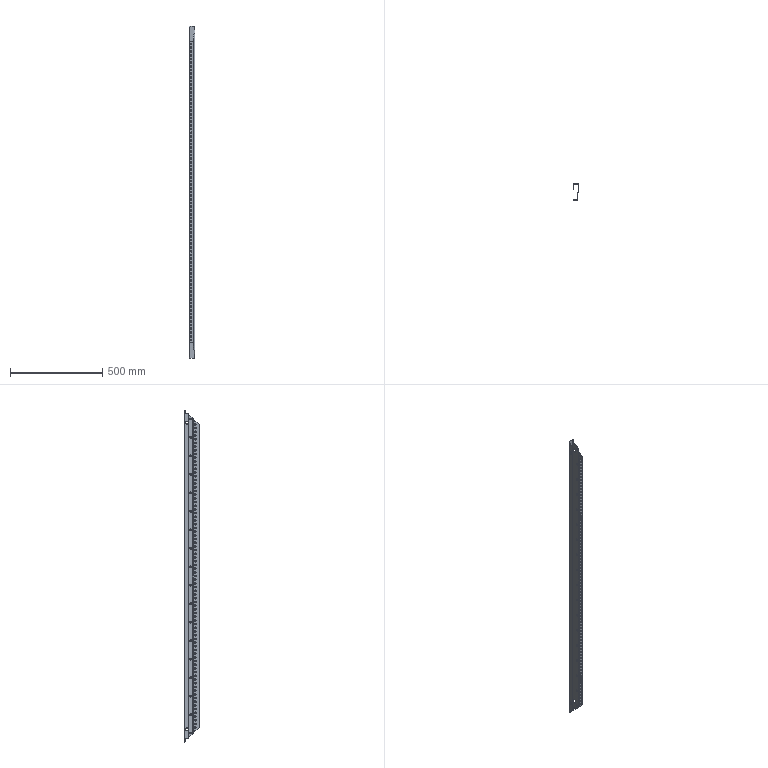Component | SolidWorks | HighVoltageCabinetFrameAssembly-1_HighVoltageCabinetVerticalFrame-2 | 1 solid | 448 faces | volume 518938 mm3 | cylinder 406 | plane 32 | spline 10 | commonest cylinder face diameters 9.2 x367 7.2 x16 22 x7 16 x6 1.473 x5 5.473 x5 | material Plain Carbon Steel